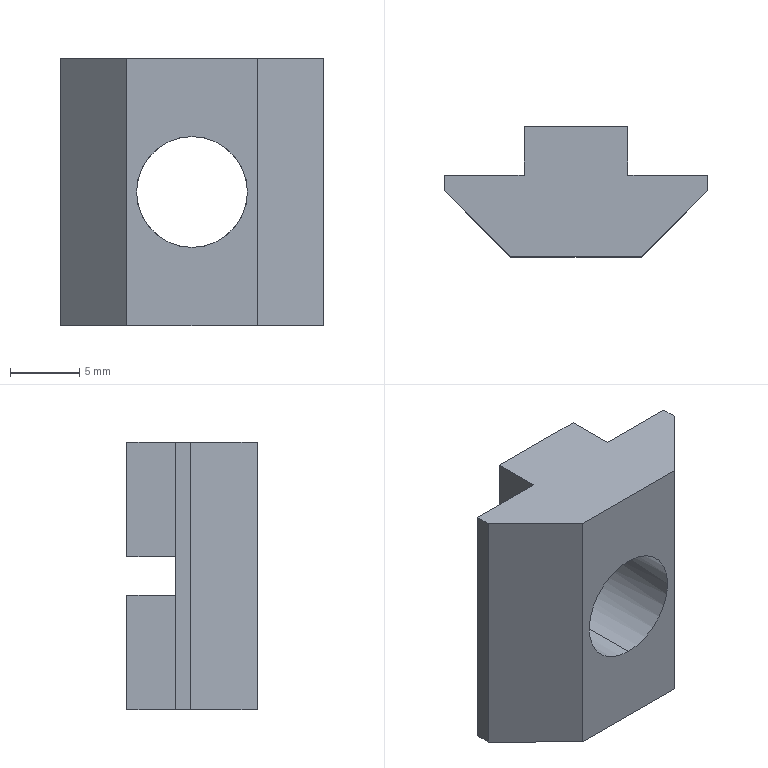Component | SolidWorks | SquareNutBlock-MC8-8-40-10 | 1 solid | 17 faces | box 19 x 9.4 x 19.3 mm | volume 1756 mm3 | plane 15 | cylinder 2 | commonest cylinder face diameters 8 x2 | material Purchased Part
build123d program:
from build123d import *

# Parameters (mm, degrees)
BOSS_EXTRUDE1_DEPTH = 9.65
M8_TAPPED_HOLE1_D   = 8


with BuildPart() as part:
    # Sketch1 → Boss-Extrude1 (new, symmetric)
    with BuildSketch(Plane.XY):
        Polygon((0, -3.75), (0, 3.75), (3.5, 3.75), (3.5, 9.5), (4.6, 9.5), (9.4, 4.7), (9.4, -4.7), (4.6, -9.5), (3.5, -9.5), (3.5, -3.75), align=None)
    extrude(amount=BOSS_EXTRUDE1_DEPTH, both=True)

    # M8 Tapped Hole1 (through all)
    with Locations(Plane(origin=(9.4, 0, 0), x_dir=(0, 0, -1), z_dir=(1, 0, 0))):
        with Locations((0, 0)):
            Hole(M8_TAPPED_HOLE1_D / 2)


solid = part.part

# Placed as in the assembly
solid = solid.moved(Location((30.4, -21, 80), (0, 0, -90)))
STEP:
#1=CARTESIAN_POINT('',(1.197,-0.8268,2.992));
#2=VERTEX_POINT('',#1);
#3=CARTESIAN_POINT('',(1.344,-0.8268,3.095));
#4=VERTEX_POINT('',#3);
#5=CARTESIAN_POINT('',(1.197,-0.8268,3.15));
#6=DIRECTION('',(0.,-1.,-0.));
#7=DIRECTION('',(0.,0.,1.));
#8=AXIS2_PLACEMENT_3D('',#5,#6,#7);
#9=CIRCLE('',#8,0.1575);
#10=EDGE_CURVE('',#2,#4,#9,.T.);
#11=ORIENTED_EDGE('',*,*,#10,.F.);
#12=CARTESIAN_POINT('',(1.197,-1.197,2.992));
#13=VERTEX_POINT('',#12);
#14=CARTESIAN_POINT('',(1.197,-1.197,2.992));
#15=DIRECTION('',(0.,-1.,-0.));
#16=VECTOR('',#15,39.37);
#17=LINE('',#14,#16);
#18=EDGE_CURVE('',#2,#13,#17,.T.);
#19=ORIENTED_EDGE('',*,*,#18,.T.);
#20=CARTESIAN_POINT('',(1.197,-1.197,3.307));
#21=VERTEX_POINT('',#20);
#22=CARTESIAN_POINT('',(1.197,-1.197,3.15));
#23=DIRECTION('',(0.,-1.,-0.));
#24=DIRECTION('',(0.,0.,1.));
#25=AXIS2_PLACEMENT_3D('',#22,#23,#24);
#26=CIRCLE('',#25,0.1575);
#27=EDGE_CURVE('',#13,#21,#26,.T.);
#28=ORIENTED_EDGE('',*,*,#27,.T.);
#29=CARTESIAN_POINT('',(1.197,-0.8268,3.307));
#30=VERTEX_POINT('',#29);
#31=CARTESIAN_POINT('',(1.197,-1.197,3.307));
#32=DIRECTION('',(0.,-1.,-0.));
#33=VECTOR('',#32,39.37);
#34=LINE('',#31,#33);
#35=EDGE_CURVE('',#30,#21,#34,.T.);
#36=ORIENTED_EDGE('',*,*,#35,.F.);
#37=CARTESIAN_POINT('',(1.344,-0.8268,3.204));
#38=VERTEX_POINT('',#37);
#39=CARTESIAN_POINT('',(1.197,-0.8268,3.15));
#40=DIRECTION('',(0.,-1.,-0.));
#41=DIRECTION('',(0.,0.,1.));
#42=AXIS2_PLACEMENT_3D('',#39,#40,#41);
#43=CIRCLE('',#42,0.1575);
#44=EDGE_CURVE('',#38,#30,#43,.T.);
#45=ORIENTED_EDGE('',*,*,#44,.F.);
#46=CARTESIAN_POINT('',(1.344,-0.9646,3.204));
#47=VERTEX_POINT('',#46);
#48=CARTESIAN_POINT('',(1.344,-1.197,3.204));
#49=DIRECTION('',(-0.,1.,0.));
#50=VECTOR('',#49,39.37);
#51=LINE('',#48,#50);
#52=EDGE_CURVE('',#47,#38,#51,.T.);
#53=ORIENTED_EDGE('',*,*,#52,.F.);
#54=CARTESIAN_POINT('',(1.344,-0.9646,3.095));
#55=VERTEX_POINT('',#54);
#56=CARTESIAN_POINT('',(1.197,-0.9646,3.15));
#57=DIRECTION('',(0.,-1.,-0.));
#58=DIRECTION('',(0.,0.,1.));
#59=AXIS2_PLACEMENT_3D('',#56,#57,#58);
#60=CIRCLE('',#59,0.1575);
#61=EDGE_CURVE('',#55,#47,#60,.T.);
#62=ORIENTED_EDGE('',*,*,#61,.F.);
#63=CARTESIAN_POINT('',(1.344,-1.197,3.095));
#64=DIRECTION('',(0.,-1.,-0.));
#65=VECTOR('',#64,39.37);
#66=LINE('',#63,#65);
#67=EDGE_CURVE('',#4,#55,#66,.T.);
#68=ORIENTED_EDGE('',*,*,#67,.F.);
#69=EDGE_LOOP('',(#11,#19,#28,#36,#45,#53,#62,#68));
#70=FACE_OUTER_BOUND('',#69,.T.);
#71=CARTESIAN_POINT('',(1.197,-1.197,3.15));
#72=DIRECTION('',(0.,-1.,-0.));
#73=DIRECTION('',(0.,0.,1.));
#74=AXIS2_PLACEMENT_3D('',#71,#72,#73);
#75=CYLINDRICAL_SURFACE('',#74,0.1575);
#76=ADVANCED_FACE('',(#70),#75,.F.);
#77=CARTESIAN_POINT('',(1.049,-0.8268,3.204));
#78=VERTEX_POINT('',#77);
#79=CARTESIAN_POINT('',(1.049,-0.8268,3.53));
#80=VERTEX_POINT('',#79);
#81=CARTESIAN_POINT('',(1.049,-0.8268,2.77));
#82=DIRECTION('',(-0.,-0.,1.));
#83=VECTOR('',#82,39.37);
#84=LINE('',#81,#83);
#85=EDGE_CURVE('',#78,#80,#84,.T.);
#86=ORIENTED_EDGE('',*,*,#85,.F.);
#87=CARTESIAN_POINT('',(1.049,-0.9646,3.204));
#88=VERTEX_POINT('',#87);
#89=CARTESIAN_POINT('',(1.049,-1.197,3.204));
#90=DIRECTION('',(0.,-1.,-0.));
#91=VECTOR('',#90,39.37);
#92=LINE('',#89,#91);
#93=EDGE_CURVE('',#78,#88,#92,.T.);
#94=ORIENTED_EDGE('',*,*,#93,.T.);
#95=CARTESIAN_POINT('',(1.049,-0.9646,3.53));
#96=VERTEX_POINT('',#95);
#97=CARTESIAN_POINT('',(1.049,-0.9646,2.77));
#98=DIRECTION('',(-0.,-0.,1.));
#99=VECTOR('',#98,39.37);
#100=LINE('',#97,#99);
#101=EDGE_CURVE('',#88,#96,#100,.T.);
#102=ORIENTED_EDGE('',*,*,#101,.T.);
#103=CARTESIAN_POINT('',(1.049,-0.8268,3.53));
#104=DIRECTION('',(-0.,1.,0.));
#105=VECTOR('',#104,39.37);
#106=LINE('',#103,#105);
#107=EDGE_CURVE('',#96,#80,#106,.T.);
#108=ORIENTED_EDGE('',*,*,#107,.T.);
#109=EDGE_LOOP('',(#86,#94,#102,#108));
#110=FACE_OUTER_BOUND('',#109,.T.);
#111=CARTESIAN_POINT('',(1.049,-0.8268,2.77));
#112=DIRECTION('',(1.,0.,0.));
#113=DIRECTION('',(-0.,-0.,1.));
#114=AXIS2_PLACEMENT_3D('',#111,#112,#113);
#115=PLANE('',#114);
#116=ADVANCED_FACE('',(#110),#115,.F.);
#117=CARTESIAN_POINT('',(1.344,-0.8268,2.77));
#118=VERTEX_POINT('',#117);
#119=CARTESIAN_POINT('',(1.344,-0.8268,2.77));
#120=DIRECTION('',(-0.,-0.,1.));
#121=VECTOR('',#120,39.37);
#122=LINE('',#119,#121);
#123=EDGE_CURVE('',#118,#4,#122,.T.);
#124=ORIENTED_EDGE('',*,*,#123,.T.);
#125=ORIENTED_EDGE('',*,*,#67,.T.);
#126=CARTESIAN_POINT('',(1.344,-0.9646,2.77));
#127=VERTEX_POINT('',#126);
#128=CARTESIAN_POINT('',(1.344,-0.9646,2.77));
#129=DIRECTION('',(-0.,-0.,1.));
#130=VECTOR('',#129,39.37);
#131=LINE('',#128,#130);
#132=EDGE_CURVE('',#127,#55,#131,.T.);
#133=ORIENTED_EDGE('',*,*,#132,.F.);
#134=CARTESIAN_POINT('',(1.344,-0.9646,2.77));
#135=DIRECTION('',(0.,-1.,-0.));
#136=VECTOR('',#135,39.37);
#137=LINE('',#134,#136);
#138=EDGE_CURVE('',#118,#127,#137,.T.);
#139=ORIENTED_EDGE('',*,*,#138,.F.);
#140=EDGE_LOOP('',(#124,#125,#133,#139));
#141=FACE_OUTER_BOUND('',#140,.T.);
#142=CARTESIAN_POINT('',(1.344,-0.9646,2.77));
#143=DIRECTION('',(-1.,-0.,-0.));
#144=DIRECTION('',(0.,0.,-1.));
#145=AXIS2_PLACEMENT_3D('',#142,#143,#144);
#146=PLANE('',#145);
#147=ADVANCED_FACE('',(#141),#146,.F.);
#148=CARTESIAN_POINT('',(1.049,-0.8268,2.77));
#149=VERTEX_POINT('',#148);
#150=CARTESIAN_POINT('',(1.049,-0.8268,3.095));
#151=VERTEX_POINT('',#150);
#152=CARTESIAN_POINT('',(1.049,-0.8268,2.77));
#153=DIRECTION('',(-0.,-0.,1.));
#154=VECTOR('',#153,39.37);
#155=LINE('',#152,#154);
#156=EDGE_CURVE('',#149,#151,#155,.T.);
#157=ORIENTED_EDGE('',*,*,#156,.T.);
#158=CARTESIAN_POINT('',(1.197,-0.8268,3.15));
#159=DIRECTION('',(0.,-1.,-0.));
#160=DIRECTION('',(0.,0.,1.));
#161=AXIS2_PLACEMENT_3D('',#158,#159,#160);
#162=CIRCLE('',#161,0.1575);
#163=EDGE_CURVE('',#151,#2,#162,.T.);
#164=ORIENTED_EDGE('',*,*,#163,.T.);
#165=ORIENTED_EDGE('',*,*,#10,.T.);
#166=ORIENTED_EDGE('',*,*,#123,.F.);
#167=CARTESIAN_POINT('',(1.344,-0.8268,2.77));
#168=DIRECTION('',(1.,0.,0.));
#169=VECTOR('',#168,39.37);
#170=LINE('',#167,#169);
#171=EDGE_CURVE('',#149,#118,#170,.T.);
#172=ORIENTED_EDGE('',*,*,#171,.F.);
#173=EDGE_LOOP('',(#157,#164,#165,#166,#172));
#174=FACE_OUTER_BOUND('',#173,.T.);
#175=CARTESIAN_POINT('',(1.344,-0.8268,2.77));
#176=DIRECTION('',(0.,-1.,0.));
#177=DIRECTION('',(-0.,-0.,1.));
#178=AXIS2_PLACEMENT_3D('',#175,#176,#177);
#179=PLANE('',#178);
#180=ADVANCED_FACE('',(#174),#179,.F.);
#181=CARTESIAN_POINT('',(1.344,-0.9646,3.53));
#182=VERTEX_POINT('',#181);
#183=CARTESIAN_POINT('',(1.344,-0.9646,2.77));
#184=DIRECTION('',(-0.,-0.,1.));
#185=VECTOR('',#184,39.37);
#186=LINE('',#183,#185);
#187=EDGE_CURVE('',#47,#182,#186,.T.);
#188=ORIENTED_EDGE('',*,*,#187,.F.);
#189=ORIENTED_EDGE('',*,*,#52,.T.);
#190=CARTESIAN_POINT('',(1.344,-0.8268,3.53));
#191=VERTEX_POINT('',#190);
#192=CARTESIAN_POINT('',(1.344,-0.8268,2.77));
#193=DIRECTION('',(-0.,-0.,1.));
#194=VECTOR('',#193,39.37);
#195=LINE('',#192,#194);
#196=EDGE_CURVE('',#38,#191,#195,.T.);
#197=ORIENTED_EDGE('',*,*,#196,.T.);
#198=CARTESIAN_POINT('',(1.344,-0.9646,3.53));
#199=DIRECTION('',(0.,-1.,-0.));
#200=VECTOR('',#199,39.37);
#201=LINE('',#198,#200);
#202=EDGE_CURVE('',#191,#182,#201,.T.);
#203=ORIENTED_EDGE('',*,*,#202,.T.);
#204=EDGE_LOOP('',(#188,#189,#197,#203));
#205=FACE_OUTER_BOUND('',#204,.T.);
#206=CARTESIAN_POINT('',(1.344,-0.9646,2.77));
#207=DIRECTION('',(-1.,-0.,-0.));
#208=DIRECTION('',(0.,0.,-1.));
#209=AXIS2_PLACEMENT_3D('',#206,#207,#208);
#210=PLANE('',#209);
#211=ADVANCED_FACE('',(#205),#210,.F.);
#212=ORIENTED_EDGE('',*,*,#132,.T.);
#213=ORIENTED_EDGE('',*,*,#61,.T.);
#214=ORIENTED_EDGE('',*,*,#187,.T.);
#215=CARTESIAN_POINT('',(1.571,-0.9646,3.53));
#216=VERTEX_POINT('',#215);
#217=CARTESIAN_POINT('',(1.571,-0.9646,3.53));
#218=DIRECTION('',(1.,0.,0.));
#219=VECTOR('',#218,39.37);
#220=LINE('',#217,#219);
#221=EDGE_CURVE('',#182,#216,#220,.T.);
#222=ORIENTED_EDGE('',*,*,#221,.T.);
#223=CARTESIAN_POINT('',(1.571,-0.9646,2.77));
#224=VERTEX_POINT('',#223);
#225=CARTESIAN_POINT('',(1.571,-0.9646,2.77));
#226=DIRECTION('',(-0.,-0.,1.));
#227=VECTOR('',#226,39.37);
#228=LINE('',#225,#227);
#229=EDGE_CURVE('',#224,#216,#228,.T.);
#230=ORIENTED_EDGE('',*,*,#229,.F.);
#231=CARTESIAN_POINT('',(1.571,-0.9646,2.77));
#232=DIRECTION('',(1.,0.,0.));
#233=VECTOR('',#232,39.37);
#234=LINE('',#231,#233);
#235=EDGE_CURVE('',#127,#224,#234,.T.);
#236=ORIENTED_EDGE('',*,*,#235,.F.);
#237=EDGE_LOOP('',(#212,#213,#214,#222,#230,#236));
#238=FACE_OUTER_BOUND('',#237,.T.);
#239=CARTESIAN_POINT('',(1.571,-0.9646,2.77));
#240=DIRECTION('',(0.,-1.,0.));
#241=DIRECTION('',(-0.,-0.,1.));
#242=AXIS2_PLACEMENT_3D('',#239,#240,#241);
#243=PLANE('',#242);
#244=ADVANCED_FACE('',(#238),#243,.F.);
#245=CARTESIAN_POINT('',(1.571,-1.008,3.53));
#246=VERTEX_POINT('',#245);
#247=CARTESIAN_POINT('',(1.571,-1.008,3.53));
#248=DIRECTION('',(0.,-1.,-0.));
#249=VECTOR('',#248,39.37);
#250=LINE('',#247,#249);
#251=EDGE_CURVE('',#216,#246,#250,.T.);
#252=ORIENTED_EDGE('',*,*,#251,.T.);
#253=CARTESIAN_POINT('',(1.571,-1.008,2.77));
#254=VERTEX_POINT('',#253);
#255=CARTESIAN_POINT('',(1.571,-1.008,2.77));
#256=DIRECTION('',(-0.,-0.,1.));
#257=VECTOR('',#256,39.37);
#258=LINE('',#255,#257);
#259=EDGE_CURVE('',#254,#246,#258,.T.);
#260=ORIENTED_EDGE('',*,*,#259,.F.);
#261=CARTESIAN_POINT('',(1.571,-1.008,2.77));
#262=DIRECTION('',(0.,-1.,-0.));
#263=VECTOR('',#262,39.37);
#264=LINE('',#261,#263);
#265=EDGE_CURVE('',#224,#254,#264,.T.);
#266=ORIENTED_EDGE('',*,*,#265,.F.);
#267=ORIENTED_EDGE('',*,*,#229,.T.);
#268=EDGE_LOOP('',(#252,#260,#266,#267));
#269=FACE_OUTER_BOUND('',#268,.T.);
#270=CARTESIAN_POINT('',(1.571,-1.008,2.77));
#271=DIRECTION('',(-1.,-0.,-0.));
#272=DIRECTION('',(0.,0.,-1.));
#273=AXIS2_PLACEMENT_3D('',#270,#271,#272);
#274=PLANE('',#273);
#275=ADVANCED_FACE('',(#269),#274,.F.);
#276=CARTESIAN_POINT('',(1.382,-1.197,3.53));
#277=VERTEX_POINT('',#276);
#278=CARTESIAN_POINT('',(1.382,-1.197,3.53));
#279=DIRECTION('',(-0.7071,-0.7071,-0.));
#280=VECTOR('',#279,39.37);
#281=LINE('',#278,#280);
#282=EDGE_CURVE('',#246,#277,#281,.T.);
#283=ORIENTED_EDGE('',*,*,#282,.T.);
#284=CARTESIAN_POINT('',(1.382,-1.197,2.77));
#285=VERTEX_POINT('',#284);
#286=CARTESIAN_POINT('',(1.382,-1.197,2.77));
#287=DIRECTION('',(-0.,-0.,1.));
#288=VECTOR('',#287,39.37);
#289=LINE('',#286,#288);
#290=EDGE_CURVE('',#285,#277,#289,.T.);
#291=ORIENTED_EDGE('',*,*,#290,.F.);
#292=CARTESIAN_POINT('',(1.382,-1.197,2.77));
#293=DIRECTION('',(-0.7071,-0.7071,-0.));
#294=VECTOR('',#293,39.37);
#295=LINE('',#292,#294);
#296=EDGE_CURVE('',#254,#285,#295,.T.);
#297=ORIENTED_EDGE('',*,*,#296,.F.);
#298=ORIENTED_EDGE('',*,*,#259,.T.);
#299=EDGE_LOOP('',(#283,#291,#297,#298));
#300=FACE_OUTER_BOUND('',#299,.T.);
#301=CARTESIAN_POINT('',(1.382,-1.197,2.77));
#302=DIRECTION('',(-0.7071,0.7071,-0.));
#303=DIRECTION('',(0.7071,0.7071,0.));
#304=AXIS2_PLACEMENT_3D('',#301,#302,#303);
#305=PLANE('',#304);
#306=ADVANCED_FACE('',(#300),#305,.F.);
#307=CARTESIAN_POINT('',(1.197,-1.197,3.15));
#308=DIRECTION('',(0.,-1.,-0.));
#309=DIRECTION('',(0.,0.,1.));
#310=AXIS2_PLACEMENT_3D('',#307,#308,#309);
#311=CIRCLE('',#310,0.1575);
#312=EDGE_CURVE('',#21,#13,#311,.T.);
#313=ORIENTED_EDGE('',*,*,#312,.F.);
#314=ORIENTED_EDGE('',*,*,#27,.F.);
#315=EDGE_LOOP('',(#313,#314));
#316=FACE_BOUND('',#315,.T.);
#317=CARTESIAN_POINT('',(1.012,-1.197,3.53));
#318=VERTEX_POINT('',#317);
#319=CARTESIAN_POINT('',(1.012,-1.197,3.53));
#320=DIRECTION('',(-1.,-0.,-0.));
#321=VECTOR('',#320,39.37);
#322=LINE('',#319,#321);
#323=EDGE_CURVE('',#277,#318,#322,.T.);
#324=ORIENTED_EDGE('',*,*,#323,.T.);
#325=CARTESIAN_POINT('',(1.012,-1.197,2.77));
#326=VERTEX_POINT('',#325);
#327=CARTESIAN_POINT('',(1.012,-1.197,2.77));
#328=DIRECTION('',(-0.,-0.,1.));
#329=VECTOR('',#328,39.37);
#330=LINE('',#327,#329);
#331=EDGE_CURVE('',#326,#318,#330,.T.);
#332=ORIENTED_EDGE('',*,*,#331,.F.);
#333=CARTESIAN_POINT('',(1.012,-1.197,2.77));
#334=DIRECTION('',(-1.,-0.,-0.));
#335=VECTOR('',#334,39.37);
#336=LINE('',#333,#335);
#337=EDGE_CURVE('',#285,#326,#336,.T.);
#338=ORIENTED_EDGE('',*,*,#337,.F.);
#339=ORIENTED_EDGE('',*,*,#290,.T.);
#340=EDGE_LOOP('',(#324,#332,#338,#339));
#341=FACE_OUTER_BOUND('',#340,.T.);
#342=CARTESIAN_POINT('',(1.012,-1.197,2.77));
#343=DIRECTION('',(-0.,1.,-0.));
#344=DIRECTION('',(0.,0.,-1.));
#345=AXIS2_PLACEMENT_3D('',#342,#343,#344);
#346=PLANE('',#345);
#347=ADVANCED_FACE('',(#316,#341),#346,.F.);
#348=CARTESIAN_POINT('',(0.8228,-1.008,3.53));
#349=VERTEX_POINT('',#348);
#350=CARTESIAN_POINT('',(0.8228,-1.008,3.53));
#351=DIRECTION('',(-0.7071,0.7071,-0.));
#352=VECTOR('',#351,39.37);
#353=LINE('',#350,#352);
#354=EDGE_CURVE('',#318,#349,#353,.T.);
#355=ORIENTED_EDGE('',*,*,#354,.T.);
#356=CARTESIAN_POINT('',(0.8228,-1.008,2.77));
#357=VERTEX_POINT('',#356);
#358=CARTESIAN_POINT('',(0.8228,-1.008,2.77));
#359=DIRECTION('',(-0.,-0.,1.));
#360=VECTOR('',#359,39.37);
#361=LINE('',#358,#360);
#362=EDGE_CURVE('',#357,#349,#361,.T.);
#363=ORIENTED_EDGE('',*,*,#362,.F.);
#364=CARTESIAN_POINT('',(0.8228,-1.008,2.77));
#365=DIRECTION('',(-0.7071,0.7071,-0.));
#366=VECTOR('',#365,39.37);
#367=LINE('',#364,#366);
#368=EDGE_CURVE('',#326,#357,#367,.T.);
#369=ORIENTED_EDGE('',*,*,#368,.F.);
#370=ORIENTED_EDGE('',*,*,#331,.T.);
#371=EDGE_LOOP('',(#355,#363,#369,#370));
#372=FACE_OUTER_BOUND('',#371,.T.);
#373=CARTESIAN_POINT('',(0.8228,-1.008,2.77));
#374=DIRECTION('',(0.7071,0.7071,0.));
#375=DIRECTION('',(0.7071,-0.7071,0.));
#376=AXIS2_PLACEMENT_3D('',#373,#374,#375);
#377=PLANE('',#376);
#378=ADVANCED_FACE('',(#372),#377,.F.);
#379=CARTESIAN_POINT('',(0.8228,-0.9646,3.53));
#380=VERTEX_POINT('',#379);
#381=CARTESIAN_POINT('',(0.8228,-0.9646,3.53));
#382=DIRECTION('',(-0.,1.,0.));
#383=VECTOR('',#382,39.37);
#384=LINE('',#381,#383);
#385=EDGE_CURVE('',#349,#380,#384,.T.);
#386=ORIENTED_EDGE('',*,*,#385,.T.);
#387=CARTESIAN_POINT('',(0.8228,-0.9646,2.77));
#388=VERTEX_POINT('',#387);
#389=CARTESIAN_POINT('',(0.8228,-0.9646,2.77));
#390=DIRECTION('',(-0.,-0.,1.));
#391=VECTOR('',#390,39.37);
#392=LINE('',#389,#391);
#393=EDGE_CURVE('',#388,#380,#392,.T.);
#394=ORIENTED_EDGE('',*,*,#393,.F.);
#395=CARTESIAN_POINT('',(0.8228,-0.9646,2.77));
#396=DIRECTION('',(-0.,1.,0.));
#397=VECTOR('',#396,39.37);
#398=LINE('',#395,#397);
#399=EDGE_CURVE('',#357,#388,#398,.T.);
#400=ORIENTED_EDGE('',*,*,#399,.F.);
#401=ORIENTED_EDGE('',*,*,#362,.T.);
#402=EDGE_LOOP('',(#386,#394,#400,#401));
#403=FACE_OUTER_BOUND('',#402,.T.);
#404=CARTESIAN_POINT('',(0.8228,-0.9646,2.77));
#405=DIRECTION('',(1.,0.,0.));
#406=DIRECTION('',(-0.,-0.,1.));
#407=AXIS2_PLACEMENT_3D('',#404,#405,#406);
#408=PLANE('',#407);
#409=ADVANCED_FACE('',(#403),#408,.F.);
#410=ORIENTED_EDGE('',*,*,#101,.F.);
#411=CARTESIAN_POINT('',(1.049,-0.9646,3.095));
#412=VERTEX_POINT('',#411);
#413=CARTESIAN_POINT('',(1.197,-0.9646,3.15));
#414=DIRECTION('',(0.,-1.,-0.));
#415=DIRECTION('',(0.,0.,1.));
#416=AXIS2_PLACEMENT_3D('',#413,#414,#415);
#417=CIRCLE('',#416,0.1575);
#418=EDGE_CURVE('',#88,#412,#417,.T.);
#419=ORIENTED_EDGE('',*,*,#418,.T.);
#420=CARTESIAN_POINT('',(1.049,-0.9646,2.77));
#421=VERTEX_POINT('',#420);
#422=CARTESIAN_POINT('',(1.049,-0.9646,2.77));
#423=DIRECTION('',(-0.,-0.,1.));
#424=VECTOR('',#423,39.37);
#425=LINE('',#422,#424);
#426=EDGE_CURVE('',#421,#412,#425,.T.);
#427=ORIENTED_EDGE('',*,*,#426,.F.);
#428=CARTESIAN_POINT('',(1.049,-0.9646,2.77));
#429=DIRECTION('',(1.,0.,0.));
#430=VECTOR('',#429,39.37);
#431=LINE('',#428,#430);
#432=EDGE_CURVE('',#388,#421,#431,.T.);
#433=ORIENTED_EDGE('',*,*,#432,.F.);
#434=ORIENTED_EDGE('',*,*,#393,.T.);
#435=CARTESIAN_POINT('',(1.049,-0.9646,3.53));
#436=DIRECTION('',(1.,0.,0.));
#437=VECTOR('',#436,39.37);
#438=LINE('',#435,#437);
#439=EDGE_CURVE('',#380,#96,#438,.T.);
#440=ORIENTED_EDGE('',*,*,#439,.T.);
#441=EDGE_LOOP('',(#410,#419,#427,#433,#434,#440));
#442=FACE_OUTER_BOUND('',#441,.T.);
#443=CARTESIAN_POINT('',(1.049,-0.9646,2.77));
#444=DIRECTION('',(0.,-1.,0.));
#445=DIRECTION('',(-0.,-0.,1.));
#446=AXIS2_PLACEMENT_3D('',#443,#444,#445);
#447=PLANE('',#446);
#448=ADVANCED_FACE('',(#442),#447,.F.);
#449=ORIENTED_EDGE('',*,*,#426,.T.);
#450=CARTESIAN_POINT('',(1.049,-1.197,3.095));
#451=DIRECTION('',(-0.,1.,0.));
#452=VECTOR('',#451,39.37);
#453=LINE('',#450,#452);
#454=EDGE_CURVE('',#412,#151,#453,.T.);
#455=ORIENTED_EDGE('',*,*,#454,.T.);
#456=ORIENTED_EDGE('',*,*,#156,.F.);
#457=CARTESIAN_POINT('',(1.049,-0.8268,2.77));
#458=DIRECTION('',(-0.,1.,0.));
#459=VECTOR('',#458,39.37);
#460=LINE('',#457,#459);
#461=EDGE_CURVE('',#421,#149,#460,.T.);
#462=ORIENTED_EDGE('',*,*,#461,.F.);
#463=EDGE_LOOP('',(#449,#455,#456,#462));
#464=FACE_OUTER_BOUND('',#463,.T.);
#465=CARTESIAN_POINT('',(1.049,-0.8268,2.77));
#466=DIRECTION('',(1.,0.,0.));
#467=DIRECTION('',(-0.,-0.,1.));
#468=AXIS2_PLACEMENT_3D('',#465,#466,#467);
#469=PLANE('',#468);
#470=ADVANCED_FACE('',(#464),#469,.F.);
#471=ORIENTED_EDGE('',*,*,#196,.F.);
#472=ORIENTED_EDGE('',*,*,#44,.T.);
#473=CARTESIAN_POINT('',(1.197,-0.8268,3.15));
#474=DIRECTION('',(0.,-1.,-0.));
#475=DIRECTION('',(0.,0.,1.));
#476=AXIS2_PLACEMENT_3D('',#473,#474,#475);
#477=CIRCLE('',#476,0.1575);
#478=EDGE_CURVE('',#30,#78,#477,.T.);
#479=ORIENTED_EDGE('',*,*,#478,.T.);
#480=ORIENTED_EDGE('',*,*,#85,.T.);
#481=CARTESIAN_POINT('',(1.344,-0.8268,3.53));
#482=DIRECTION('',(1.,0.,0.));
#483=VECTOR('',#482,39.37);
#484=LINE('',#481,#483);
#485=EDGE_CURVE('',#80,#191,#484,.T.);
#486=ORIENTED_EDGE('',*,*,#485,.T.);
#487=EDGE_LOOP('',(#471,#472,#479,#480,#486));
#488=FACE_OUTER_BOUND('',#487,.T.);
#489=CARTESIAN_POINT('',(1.344,-0.8268,2.77));
#490=DIRECTION('',(0.,-1.,0.));
#491=DIRECTION('',(-0.,-0.,1.));
#492=AXIS2_PLACEMENT_3D('',#489,#490,#491);
#493=PLANE('',#492);
#494=ADVANCED_FACE('',(#488),#493,.F.);
#495=ORIENTED_EDGE('',*,*,#138,.T.);
#496=ORIENTED_EDGE('',*,*,#235,.T.);
#497=ORIENTED_EDGE('',*,*,#265,.T.);
#498=ORIENTED_EDGE('',*,*,#296,.T.);
#499=ORIENTED_EDGE('',*,*,#337,.T.);
#500=ORIENTED_EDGE('',*,*,#368,.T.);
#501=ORIENTED_EDGE('',*,*,#399,.T.);
#502=ORIENTED_EDGE('',*,*,#432,.T.);
#503=ORIENTED_EDGE('',*,*,#461,.T.);
#504=ORIENTED_EDGE('',*,*,#171,.T.);
#505=EDGE_LOOP('',(#495,#496,#497,#498,#499,#500,#501,#502,#503,#504));
#506=FACE_OUTER_BOUND('',#505,.T.);
#507=CARTESIAN_POINT('',(1.197,-0.8268,2.77));
#508=DIRECTION('',(-0.,-0.,1.));
#509=DIRECTION('',(-0.,1.,0.));
#510=AXIS2_PLACEMENT_3D('',#507,#508,#509);
#511=PLANE('',#510);
#512=ADVANCED_FACE('',(#506),#511,.F.);
#513=ORIENTED_EDGE('',*,*,#202,.F.);
#514=ORIENTED_EDGE('',*,*,#485,.F.);
#515=ORIENTED_EDGE('',*,*,#107,.F.);
#516=ORIENTED_EDGE('',*,*,#439,.F.);
#517=ORIENTED_EDGE('',*,*,#385,.F.);
#518=ORIENTED_EDGE('',*,*,#354,.F.);
#519=ORIENTED_EDGE('',*,*,#323,.F.);
#520=ORIENTED_EDGE('',*,*,#282,.F.);
#521=ORIENTED_EDGE('',*,*,#251,.F.);
#522=ORIENTED_EDGE('',*,*,#221,.F.);
#523=EDGE_LOOP('',(#513,#514,#515,#516,#517,#518,#519,#520,#521,#522));
#524=FACE_OUTER_BOUND('',#523,.T.);
#525=CARTESIAN_POINT('',(1.197,-0.8268,3.53));
#526=DIRECTION('',(-0.,-0.,1.));
#527=DIRECTION('',(-0.,1.,0.));
#528=AXIS2_PLACEMENT_3D('',#525,#526,#527);
#529=PLANE('',#528);
#530=ADVANCED_FACE('',(#524),#529,.T.);
#531=ORIENTED_EDGE('',*,*,#18,.F.);
#532=ORIENTED_EDGE('',*,*,#163,.F.);
#533=ORIENTED_EDGE('',*,*,#454,.F.);
#534=ORIENTED_EDGE('',*,*,#418,.F.);
#535=ORIENTED_EDGE('',*,*,#93,.F.);
#536=ORIENTED_EDGE('',*,*,#478,.F.);
#537=ORIENTED_EDGE('',*,*,#35,.T.);
#538=ORIENTED_EDGE('',*,*,#312,.T.);
#539=EDGE_LOOP('',(#531,#532,#533,#534,#535,#536,#537,#538));
#540=FACE_OUTER_BOUND('',#539,.T.);
#541=CARTESIAN_POINT('',(1.197,-1.197,3.15));
#542=DIRECTION('',(0.,-1.,-0.));
#543=DIRECTION('',(0.,0.,1.));
#544=AXIS2_PLACEMENT_3D('',#541,#542,#543);
#545=CYLINDRICAL_SURFACE('',#544,0.1575);
#546=ADVANCED_FACE('',(#540),#545,.F.);
#547=CLOSED_SHELL('',(#76,#116,#147,#180,#211,#244,#275,#306,#347,#378,#409,#448,#470,#494,#512,#530,#546));
#548=MANIFOLD_SOLID_BREP('',#547);
#549=CARTESIAN_POINT('',(0.,0.,0.));
#550=DIRECTION('',(0.,0.,1.));
#551=DIRECTION('',(1.,0.,0.));
#552=AXIS2_PLACEMENT_3D('',#549,#550,#551);
#553=(LENGTH_UNIT()NAMED_UNIT(*)SI_UNIT($,.METRE.));
#554=LENGTH_MEASURE_WITH_UNIT(LENGTH_MEASURE(0.0254),#553);
#555=DIMENSIONAL_EXPONENTS(1.,0.,0.,0.,0.,0.,0.);
#556=(CONVERSION_BASED_UNIT('',#554)LENGTH_UNIT()NAMED_UNIT(#555));
#557=UNCERTAINTY_MEASURE_WITH_UNIT(LENGTH_MEASURE(0.00001),#556,'','');
#558=(NAMED_UNIT(*)PLANE_ANGLE_UNIT()SI_UNIT($,.RADIAN.));
#559=(NAMED_UNIT(*)SI_UNIT($,.STERADIAN.)SOLID_ANGLE_UNIT());
#560=(GEOMETRIC_REPRESENTATION_CONTEXT(3)GLOBAL_UNCERTAINTY_ASSIGNED_CONTEXT((#557))GLOBAL_UNIT_ASSIGNED_CONTEXT((#556,#558,#559))REPRESENTATION_CONTEXT('',''));
#561=ADVANCED_BREP_SHAPE_REPRESENTATION('',(#548,#552),#560);
#562=COLOUR_RGB('',0.7922,0.8196,0.9333);
#563=FILL_AREA_STYLE_COLOUR('',#562);
#564=FILL_AREA_STYLE('',(#563));
#565=SURFACE_STYLE_FILL_AREA(#564);
#566=SURFACE_SIDE_STYLE('',(#565));
#567=SURFACE_STYLE_USAGE(.BOTH.,#566);
#568=PRESENTATION_STYLE_ASSIGNMENT((#567));
#569=STYLED_ITEM('',(#568),#548);
#570=(LENGTH_UNIT()NAMED_UNIT(*)SI_UNIT($,.METRE.));
#571=LENGTH_MEASURE_WITH_UNIT(LENGTH_MEASURE(0.0254),#570);
#572=DIMENSIONAL_EXPONENTS(1.,0.,0.,0.,0.,0.,0.);
#573=(CONVERSION_BASED_UNIT('',#571)LENGTH_UNIT()NAMED_UNIT(#572));
#574=UNCERTAINTY_MEASURE_WITH_UNIT(LENGTH_MEASURE(0.00001),#573,'','');
#575=(NAMED_UNIT(*)PLANE_ANGLE_UNIT()SI_UNIT($,.RADIAN.));
#576=(NAMED_UNIT(*)SI_UNIT($,.STERADIAN.)SOLID_ANGLE_UNIT());
#577=(GEOMETRIC_REPRESENTATION_CONTEXT(3)GLOBAL_UNCERTAINTY_ASSIGNED_CONTEXT((#574))GLOBAL_UNIT_ASSIGNED_CONTEXT((#573,#575,#576))REPRESENTATION_CONTEXT('',''));
#578=MECHANICAL_DESIGN_GEOMETRIC_PRESENTATION_REPRESENTATION('',(#569),#577);
#579=PRESENTATION_LAYER_ASSIGNMENT('','',(#569));